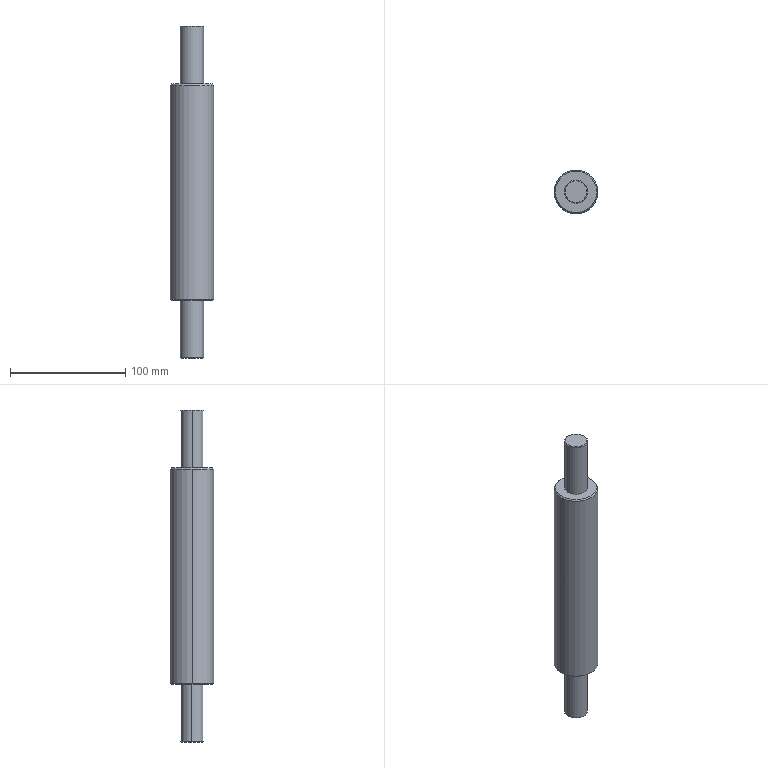Component | SolidWorks | CuttingMotorFixedAxis-1 | 1 solid | 18 faces | box 38 x 38 x 288 mm | volume 244475 mm3 | cone 8 | cylinder 6 | plane 4 | commonest cylinder face diameters 20 x4 38 x2
build123d program:
from build123d import *
from OCP.BRepFilletAPI import BRepFilletAPI_MakeChamfer

# Parameters (mm, degrees)
CHAMFER1_SIZE  = 0.5
CHAMFER2_SIZE  = 1
CHAMFER2_SIZE2 = 1.192


with BuildPart() as part:
    # Sketch1 → Revolve1 (revolve)
    with BuildSketch(Plane.XY, mode=Mode.PRIVATE) as revolve1_sk:
        Polygon((0, 0), (0, 10), (50, 10), (50, 19), (238, 19), (238, 10), (288, 10), (288, 0), align=None)
    revolve(revolve1_sk.sketch.rotate(Axis((-313.729, 0, 0), (1, 0, 0)), 90), axis=Axis((-313.729, 0, 0), (1, 0, 0)))

    # Chamfer1
    chamfer1_edges = [part.edges().sort_by_distance(p)[0] for p in [
        (288, 0, -10),
        (0, 0, -10),
    ]]
    chamfer(chamfer1_edges, length=CHAMFER1_SIZE)

    # Chamfer2: one chamfer whose edges measure the first distance from different faces: ONE call of the kernel's chamfer builder (chamfer() names one face for all edges)
    chamfer2_edges_1 = [part.edges().sort_by_distance(p)[0] for p in [
        (238, 0, -19),
    ]]
    chamfer2_side_1 = [part.faces().sort_by_distance(p)[0] for p in [
        (238, 0, -18.463),
    ]]
    chamfer2_edges_2 = [part.edges().sort_by_distance(p)[0] for p in [
        (50, 0, -19),
    ]]
    chamfer2_side_2 = [part.faces().sort_by_distance(p)[0] for p in [
        (144, 0, -19),
    ]]
    chamfer2 = BRepFilletAPI_MakeChamfer(part.part.solid().wrapped)
    for e in chamfer2_edges_1:
        chamfer2.Add(CHAMFER2_SIZE, CHAMFER2_SIZE2, e.wrapped, chamfer2_side_1[0].wrapped)  # the first distance lies on this face
    for e in chamfer2_edges_2:
        chamfer2.Add(CHAMFER2_SIZE, CHAMFER2_SIZE2, e.wrapped, chamfer2_side_2[0].wrapped)  # the first distance lies on this face
    add(Compound.cast(chamfer2.Shape()), mode=Mode.REPLACE)


solid = part.part

# Placed as in the assembly
solid = solid.moved(Location((-22.772, -46.766, 756), (0, -90, 0)))
STEP:
#1=COLOUR_RGB('',0.7922,0.8196,0.9333);
#2=FILL_AREA_STYLE_COLOUR('',#1);
#3=FILL_AREA_STYLE('',(#2));
#4=SURFACE_STYLE_FILL_AREA(#3);
#5=SURFACE_SIDE_STYLE('',(#4));
#6=SURFACE_STYLE_USAGE(.BOTH.,#5);
#7=PRESENTATION_STYLE_ASSIGNMENT((#6));
#8=CARTESIAN_POINT('',(-1.598,-1.841,31.732));
#9=VERTEX_POINT('',#8);
#10=CARTESIAN_POINT('',(-0.1954,-1.841,31.732));
#11=VERTEX_POINT('',#10);
#12=CARTESIAN_POINT('',(-0.8965,-1.841,31.732));
#13=DIRECTION('',(-0.,0.,-1.));
#14=DIRECTION('',(1.,0.,0.));
#15=AXIS2_PLACEMENT_3D('',#12,#13,#14);
#16=CIRCLE('',#15,0.7011);
#17=EDGE_CURVE('',#9,#11,#16,.T.);
#18=ORIENTED_EDGE('',*,*,#17,.F.);
#19=CARTESIAN_POINT('',(-1.645,-1.841,31.772));
#20=VERTEX_POINT('',#19);
#21=CARTESIAN_POINT('',(-1.598,-1.841,31.732));
#22=DIRECTION('',(-0.766,-0.,0.6428));
#23=VECTOR('',#22,39.37);
#24=LINE('',#21,#23);
#25=EDGE_CURVE('',#9,#20,#24,.T.);
#26=ORIENTED_EDGE('',*,*,#25,.T.);
#27=CARTESIAN_POINT('',(-0.1485,-1.841,31.772));
#28=VERTEX_POINT('',#27);
#29=CARTESIAN_POINT('',(-0.8965,-1.841,31.772));
#30=DIRECTION('',(0.,-0.,1.));
#31=DIRECTION('',(1.,0.,0.));
#32=AXIS2_PLACEMENT_3D('',#29,#30,#31);
#33=CIRCLE('',#32,0.748);
#34=EDGE_CURVE('',#28,#20,#33,.T.);
#35=ORIENTED_EDGE('',*,*,#34,.F.);
#36=CARTESIAN_POINT('',(-0.1954,-1.841,31.732));
#37=DIRECTION('',(0.766,-0.,0.6428));
#38=VECTOR('',#37,39.37);
#39=LINE('',#36,#38);
#40=EDGE_CURVE('',#11,#28,#39,.T.);
#41=ORIENTED_EDGE('',*,*,#40,.F.);
#42=EDGE_LOOP('',(#18,#26,#35,#41));
#43=FACE_OUTER_BOUND('',#42,.T.);
#44=CARTESIAN_POINT('',(-0.8965,-1.841,31.732));
#45=DIRECTION('',(0.,-0.,1.));
#46=DIRECTION('',(1.,0.,0.));
#47=AXIS2_PLACEMENT_3D('',#44,#45,#46);
#48=CONICAL_SURFACE('',#47,0.7011,0.8727);
#49=ADVANCED_FACE('',(#43),#48,.T.);
#50=CARTESIAN_POINT('',(-0.1879,-1.841,39.134));
#51=VERTEX_POINT('',#50);
#52=CARTESIAN_POINT('',(-1.605,-1.841,39.134));
#53=VERTEX_POINT('',#52);
#54=CARTESIAN_POINT('',(-0.8965,-1.841,39.134));
#55=DIRECTION('',(0.,-0.,1.));
#56=DIRECTION('',(-1.,-0.,0.));
#57=AXIS2_PLACEMENT_3D('',#54,#55,#56);
#58=CIRCLE('',#57,0.7087);
#59=EDGE_CURVE('',#51,#53,#58,.T.);
#60=ORIENTED_EDGE('',*,*,#59,.F.);
#61=CARTESIAN_POINT('',(-0.1485,-1.841,39.087));
#62=VERTEX_POINT('',#61);
#63=CARTESIAN_POINT('',(-0.1485,-1.841,39.087));
#64=DIRECTION('',(0.6428,0.,-0.766));
#65=VECTOR('',#64,39.37);
#66=LINE('',#63,#65);
#67=EDGE_CURVE('',#51,#62,#66,.T.);
#68=ORIENTED_EDGE('',*,*,#67,.T.);
#69=CARTESIAN_POINT('',(-1.645,-1.841,39.087));
#70=VERTEX_POINT('',#69);
#71=CARTESIAN_POINT('',(-0.8965,-1.841,39.087));
#72=DIRECTION('',(-0.,0.,-1.));
#73=DIRECTION('',(-1.,-0.,0.));
#74=AXIS2_PLACEMENT_3D('',#71,#72,#73);
#75=CIRCLE('',#74,0.748);
#76=EDGE_CURVE('',#70,#62,#75,.T.);
#77=ORIENTED_EDGE('',*,*,#76,.F.);
#78=CARTESIAN_POINT('',(-1.645,-1.841,39.087));
#79=DIRECTION('',(-0.6428,0.,-0.766));
#80=VECTOR('',#79,39.37);
#81=LINE('',#78,#80);
#82=EDGE_CURVE('',#53,#70,#81,.T.);
#83=ORIENTED_EDGE('',*,*,#82,.F.);
#84=EDGE_LOOP('',(#60,#68,#77,#83));
#85=FACE_OUTER_BOUND('',#84,.T.);
#86=CARTESIAN_POINT('',(-0.8965,-1.841,39.087));
#87=DIRECTION('',(-0.,0.,-1.));
#88=DIRECTION('',(-1.,-0.,0.));
#89=AXIS2_PLACEMENT_3D('',#86,#87,#88);
#90=CONICAL_SURFACE('',#89,0.748,0.6981);
#91=ADVANCED_FACE('',(#85),#90,.T.);
#92=CARTESIAN_POINT('',(-1.271,-1.841,29.764));
#93=VERTEX_POINT('',#92);
#94=CARTESIAN_POINT('',(-0.5225,-1.841,29.764));
#95=VERTEX_POINT('',#94);
#96=CARTESIAN_POINT('',(-0.8965,-1.841,29.764));
#97=DIRECTION('',(-0.,0.,-1.));
#98=DIRECTION('',(1.,0.,0.));
#99=AXIS2_PLACEMENT_3D('',#96,#97,#98);
#100=CIRCLE('',#99,0.374);
#101=EDGE_CURVE('',#93,#95,#100,.T.);
#102=ORIENTED_EDGE('',*,*,#101,.F.);
#103=CARTESIAN_POINT('',(-1.29,-1.841,29.783));
#104=VERTEX_POINT('',#103);
#105=CARTESIAN_POINT('',(-1.271,-1.841,29.764));
#106=DIRECTION('',(-0.7071,-0.,0.7071));
#107=VECTOR('',#106,39.37);
#108=LINE('',#105,#107);
#109=EDGE_CURVE('',#93,#104,#108,.T.);
#110=ORIENTED_EDGE('',*,*,#109,.T.);
#111=CARTESIAN_POINT('',(-0.5028,-1.841,29.783));
#112=VERTEX_POINT('',#111);
#113=CARTESIAN_POINT('',(-0.8965,-1.841,29.783));
#114=DIRECTION('',(0.,-0.,1.));
#115=DIRECTION('',(1.,0.,0.));
#116=AXIS2_PLACEMENT_3D('',#113,#114,#115);
#117=CIRCLE('',#116,0.3937);
#118=EDGE_CURVE('',#112,#104,#117,.T.);
#119=ORIENTED_EDGE('',*,*,#118,.F.);
#120=CARTESIAN_POINT('',(-0.5225,-1.841,29.764));
#121=DIRECTION('',(0.7071,-0.,0.7071));
#122=VECTOR('',#121,39.37);
#123=LINE('',#120,#122);
#124=EDGE_CURVE('',#95,#112,#123,.T.);
#125=ORIENTED_EDGE('',*,*,#124,.F.);
#126=EDGE_LOOP('',(#102,#110,#119,#125));
#127=FACE_OUTER_BOUND('',#126,.T.);
#128=CARTESIAN_POINT('',(-0.8965,-1.841,29.764));
#129=DIRECTION('',(0.,-0.,1.));
#130=DIRECTION('',(1.,0.,0.));
#131=AXIS2_PLACEMENT_3D('',#128,#129,#130);
#132=CONICAL_SURFACE('',#131,0.374,0.7854);
#133=ADVANCED_FACE('',(#127),#132,.T.);
#134=CARTESIAN_POINT('',(-0.5225,-1.841,41.102));
#135=VERTEX_POINT('',#134);
#136=CARTESIAN_POINT('',(-1.271,-1.841,41.102));
#137=VERTEX_POINT('',#136);
#138=CARTESIAN_POINT('',(-0.8965,-1.841,41.102));
#139=DIRECTION('',(0.,-0.,1.));
#140=DIRECTION('',(-1.,0.,0.));
#141=AXIS2_PLACEMENT_3D('',#138,#139,#140);
#142=CIRCLE('',#141,0.374);
#143=EDGE_CURVE('',#135,#137,#142,.T.);
#144=ORIENTED_EDGE('',*,*,#143,.F.);
#145=CARTESIAN_POINT('',(-0.5028,-1.841,41.083));
#146=VERTEX_POINT('',#145);
#147=CARTESIAN_POINT('',(-0.5028,-1.841,41.083));
#148=DIRECTION('',(0.7071,0.,-0.7071));
#149=VECTOR('',#148,39.37);
#150=LINE('',#147,#149);
#151=EDGE_CURVE('',#135,#146,#150,.T.);
#152=ORIENTED_EDGE('',*,*,#151,.T.);
#153=CARTESIAN_POINT('',(-1.29,-1.841,41.083));
#154=VERTEX_POINT('',#153);
#155=CARTESIAN_POINT('',(-0.8965,-1.841,41.083));
#156=DIRECTION('',(-0.,0.,-1.));
#157=DIRECTION('',(-1.,0.,0.));
#158=AXIS2_PLACEMENT_3D('',#155,#156,#157);
#159=CIRCLE('',#158,0.3937);
#160=EDGE_CURVE('',#154,#146,#159,.T.);
#161=ORIENTED_EDGE('',*,*,#160,.F.);
#162=CARTESIAN_POINT('',(-1.29,-1.841,41.083));
#163=DIRECTION('',(-0.7071,0.,-0.7071));
#164=VECTOR('',#163,39.37);
#165=LINE('',#162,#164);
#166=EDGE_CURVE('',#137,#154,#165,.T.);
#167=ORIENTED_EDGE('',*,*,#166,.F.);
#168=EDGE_LOOP('',(#144,#152,#161,#167));
#169=FACE_OUTER_BOUND('',#168,.T.);
#170=CARTESIAN_POINT('',(-0.8965,-1.841,41.083));
#171=DIRECTION('',(-0.,0.,-1.));
#172=DIRECTION('',(-1.,0.,0.));
#173=AXIS2_PLACEMENT_3D('',#170,#171,#172);
#174=CONICAL_SURFACE('',#173,0.3937,0.7854);
#175=ADVANCED_FACE('',(#169),#174,.T.);
#176=ORIENTED_EDGE('',*,*,#160,.T.);
#177=CARTESIAN_POINT('',(-0.5028,-1.841,39.134));
#178=VERTEX_POINT('',#177);
#179=CARTESIAN_POINT('',(-0.5028,-1.841,17.412));
#180=DIRECTION('',(-0.,0.,-1.));
#181=VECTOR('',#180,39.37);
#182=LINE('',#179,#181);
#183=EDGE_CURVE('',#146,#178,#182,.T.);
#184=ORIENTED_EDGE('',*,*,#183,.T.);
#185=CARTESIAN_POINT('',(-1.29,-1.841,39.134));
#186=VERTEX_POINT('',#185);
#187=CARTESIAN_POINT('',(-0.8965,-1.841,39.134));
#188=DIRECTION('',(-0.,0.,-1.));
#189=DIRECTION('',(-1.,0.,0.));
#190=AXIS2_PLACEMENT_3D('',#187,#188,#189);
#191=CIRCLE('',#190,0.3937);
#192=EDGE_CURVE('',#186,#178,#191,.T.);
#193=ORIENTED_EDGE('',*,*,#192,.F.);
#194=CARTESIAN_POINT('',(-1.29,-1.841,17.412));
#195=DIRECTION('',(-0.,0.,-1.));
#196=VECTOR('',#195,39.37);
#197=LINE('',#194,#196);
#198=EDGE_CURVE('',#154,#186,#197,.T.);
#199=ORIENTED_EDGE('',*,*,#198,.F.);
#200=EDGE_LOOP('',(#176,#184,#193,#199));
#201=FACE_OUTER_BOUND('',#200,.T.);
#202=CARTESIAN_POINT('',(-0.8965,-1.841,17.412));
#203=DIRECTION('',(-0.,0.,-1.));
#204=DIRECTION('',(-1.,0.,0.));
#205=AXIS2_PLACEMENT_3D('',#202,#203,#204);
#206=CYLINDRICAL_SURFACE('',#205,0.3937);
#207=ADVANCED_FACE('',(#201),#206,.T.);
#208=ORIENTED_EDGE('',*,*,#76,.T.);
#209=CARTESIAN_POINT('',(-0.1485,-1.841,17.412));
#210=DIRECTION('',(-0.,0.,-1.));
#211=VECTOR('',#210,39.37);
#212=LINE('',#209,#211);
#213=EDGE_CURVE('',#62,#28,#212,.T.);
#214=ORIENTED_EDGE('',*,*,#213,.T.);
#215=ORIENTED_EDGE('',*,*,#34,.T.);
#216=CARTESIAN_POINT('',(-1.645,-1.841,17.412));
#217=DIRECTION('',(-0.,0.,-1.));
#218=VECTOR('',#217,39.37);
#219=LINE('',#216,#218);
#220=EDGE_CURVE('',#70,#20,#219,.T.);
#221=ORIENTED_EDGE('',*,*,#220,.F.);
#222=EDGE_LOOP('',(#208,#214,#215,#221));
#223=FACE_OUTER_BOUND('',#222,.T.);
#224=CARTESIAN_POINT('',(-0.8965,-1.841,17.412));
#225=DIRECTION('',(-0.,0.,-1.));
#226=DIRECTION('',(-1.,-0.,0.));
#227=AXIS2_PLACEMENT_3D('',#224,#225,#226);
#228=CYLINDRICAL_SURFACE('',#227,0.748);
#229=ADVANCED_FACE('',(#223),#228,.T.);
#230=CARTESIAN_POINT('',(-1.29,-1.841,31.732));
#231=VERTEX_POINT('',#230);
#232=CARTESIAN_POINT('',(-0.5028,-1.841,31.732));
#233=VERTEX_POINT('',#232);
#234=CARTESIAN_POINT('',(-0.8965,-1.841,31.732));
#235=DIRECTION('',(-0.,0.,-1.));
#236=DIRECTION('',(-1.,0.,0.));
#237=AXIS2_PLACEMENT_3D('',#234,#235,#236);
#238=CIRCLE('',#237,0.3937);
#239=EDGE_CURVE('',#231,#233,#238,.T.);
#240=ORIENTED_EDGE('',*,*,#239,.T.);
#241=CARTESIAN_POINT('',(-0.5028,-1.841,17.412));
#242=DIRECTION('',(-0.,0.,-1.));
#243=VECTOR('',#242,39.37);
#244=LINE('',#241,#243);
#245=EDGE_CURVE('',#233,#112,#244,.T.);
#246=ORIENTED_EDGE('',*,*,#245,.T.);
#247=ORIENTED_EDGE('',*,*,#118,.T.);
#248=CARTESIAN_POINT('',(-1.29,-1.841,17.412));
#249=DIRECTION('',(-0.,0.,-1.));
#250=VECTOR('',#249,39.37);
#251=LINE('',#248,#250);
#252=EDGE_CURVE('',#231,#104,#251,.T.);
#253=ORIENTED_EDGE('',*,*,#252,.F.);
#254=EDGE_LOOP('',(#240,#246,#247,#253));
#255=FACE_OUTER_BOUND('',#254,.T.);
#256=CARTESIAN_POINT('',(-0.8965,-1.841,17.412));
#257=DIRECTION('',(-0.,0.,-1.));
#258=DIRECTION('',(-1.,0.,0.));
#259=AXIS2_PLACEMENT_3D('',#256,#257,#258);
#260=CYLINDRICAL_SURFACE('',#259,0.3937);
#261=ADVANCED_FACE('',(#255),#260,.T.);
#262=CARTESIAN_POINT('',(-0.8965,-1.841,29.764));
#263=DIRECTION('',(-0.,0.,-1.));
#264=DIRECTION('',(1.,0.,0.));
#265=AXIS2_PLACEMENT_3D('',#262,#263,#264);
#266=CIRCLE('',#265,0.374);
#267=EDGE_CURVE('',#95,#93,#266,.T.);
#268=ORIENTED_EDGE('',*,*,#267,.T.);
#269=ORIENTED_EDGE('',*,*,#101,.T.);
#270=EDGE_LOOP('',(#268,#269));
#271=FACE_OUTER_BOUND('',#270,.T.);
#272=CARTESIAN_POINT('',(-0.8965,-1.841,29.764));
#273=DIRECTION('',(0.,-0.,1.));
#274=DIRECTION('',(1.,0.,-0.));
#275=AXIS2_PLACEMENT_3D('',#272,#273,#274);
#276=PLANE('',#275);
#277=ADVANCED_FACE('',(#271),#276,.F.);
#278=ORIENTED_EDGE('',*,*,#245,.F.);
#279=CARTESIAN_POINT('',(-0.8965,-1.841,31.732));
#280=DIRECTION('',(-0.,0.,-1.));
#281=DIRECTION('',(-1.,0.,0.));
#282=AXIS2_PLACEMENT_3D('',#279,#280,#281);
#283=CIRCLE('',#282,0.3937);
#284=EDGE_CURVE('',#233,#231,#283,.T.);
#285=ORIENTED_EDGE('',*,*,#284,.T.);
#286=ORIENTED_EDGE('',*,*,#252,.T.);
#287=CARTESIAN_POINT('',(-0.8965,-1.841,29.783));
#288=DIRECTION('',(0.,-0.,1.));
#289=DIRECTION('',(1.,0.,0.));
#290=AXIS2_PLACEMENT_3D('',#287,#288,#289);
#291=CIRCLE('',#290,0.3937);
#292=EDGE_CURVE('',#104,#112,#291,.T.);
#293=ORIENTED_EDGE('',*,*,#292,.T.);
#294=EDGE_LOOP('',(#278,#285,#286,#293));
#295=FACE_OUTER_BOUND('',#294,.T.);
#296=CARTESIAN_POINT('',(-0.8965,-1.841,17.412));
#297=DIRECTION('',(-0.,0.,-1.));
#298=DIRECTION('',(-1.,0.,0.));
#299=AXIS2_PLACEMENT_3D('',#296,#297,#298);
#300=CYLINDRICAL_SURFACE('',#299,0.3937);
#301=ADVANCED_FACE('',(#295),#300,.T.);
#302=CARTESIAN_POINT('',(-0.8965,-1.841,31.732));
#303=DIRECTION('',(-0.,0.,-1.));
#304=DIRECTION('',(1.,0.,0.));
#305=AXIS2_PLACEMENT_3D('',#302,#303,#304);
#306=CIRCLE('',#305,0.7011);
#307=EDGE_CURVE('',#11,#9,#306,.T.);
#308=ORIENTED_EDGE('',*,*,#307,.T.);
#309=ORIENTED_EDGE('',*,*,#17,.T.);
#310=EDGE_LOOP('',(#308,#309));
#311=FACE_OUTER_BOUND('',#310,.T.);
#312=ORIENTED_EDGE('',*,*,#239,.F.);
#313=ORIENTED_EDGE('',*,*,#284,.F.);
#314=EDGE_LOOP('',(#312,#313));
#315=FACE_BOUND('',#314,.T.);
#316=CARTESIAN_POINT('',(-0.8965,-1.447,31.732));
#317=DIRECTION('',(0.,-0.,1.));
#318=DIRECTION('',(1.,0.,-0.));
#319=AXIS2_PLACEMENT_3D('',#316,#317,#318);
#320=PLANE('',#319);
#321=ADVANCED_FACE('',(#311,#315),#320,.F.);
#322=ORIENTED_EDGE('',*,*,#213,.F.);
#323=CARTESIAN_POINT('',(-0.8965,-1.841,39.087));
#324=DIRECTION('',(-0.,0.,-1.));
#325=DIRECTION('',(-1.,-0.,0.));
#326=AXIS2_PLACEMENT_3D('',#323,#324,#325);
#327=CIRCLE('',#326,0.748);
#328=EDGE_CURVE('',#62,#70,#327,.T.);
#329=ORIENTED_EDGE('',*,*,#328,.T.);
#330=ORIENTED_EDGE('',*,*,#220,.T.);
#331=CARTESIAN_POINT('',(-0.8965,-1.841,31.772));
#332=DIRECTION('',(0.,-0.,1.));
#333=DIRECTION('',(1.,0.,0.));
#334=AXIS2_PLACEMENT_3D('',#331,#332,#333);
#335=CIRCLE('',#334,0.748);
#336=EDGE_CURVE('',#20,#28,#335,.T.);
#337=ORIENTED_EDGE('',*,*,#336,.T.);
#338=EDGE_LOOP('',(#322,#329,#330,#337));
#339=FACE_OUTER_BOUND('',#338,.T.);
#340=CARTESIAN_POINT('',(-0.8965,-1.841,17.412));
#341=DIRECTION('',(-0.,0.,-1.));
#342=DIRECTION('',(-1.,-0.,0.));
#343=AXIS2_PLACEMENT_3D('',#340,#341,#342);
#344=CYLINDRICAL_SURFACE('',#343,0.748);
#345=ADVANCED_FACE('',(#339),#344,.T.);
#346=CARTESIAN_POINT('',(-0.8965,-1.841,39.134));
#347=DIRECTION('',(0.,-0.,1.));
#348=DIRECTION('',(-1.,-0.,0.));
#349=AXIS2_PLACEMENT_3D('',#346,#347,#348);
#350=CIRCLE('',#349,0.7087);
#351=EDGE_CURVE('',#53,#51,#350,.T.);
#352=ORIENTED_EDGE('',*,*,#351,.T.);
#353=ORIENTED_EDGE('',*,*,#59,.T.);
#354=EDGE_LOOP('',(#352,#353));
#355=FACE_OUTER_BOUND('',#354,.T.);
#356=ORIENTED_EDGE('',*,*,#192,.T.);
#357=CARTESIAN_POINT('',(-0.8965,-1.841,39.134));
#358=DIRECTION('',(-0.,0.,-1.));
#359=DIRECTION('',(-1.,0.,0.));
#360=AXIS2_PLACEMENT_3D('',#357,#358,#359);
#361=CIRCLE('',#360,0.3937);
#362=EDGE_CURVE('',#178,#186,#361,.T.);
#363=ORIENTED_EDGE('',*,*,#362,.T.);
#364=EDGE_LOOP('',(#356,#363));
#365=FACE_BOUND('',#364,.T.);
#366=CARTESIAN_POINT('',(-0.8965,-1.093,39.134));
#367=DIRECTION('',(-0.,0.,-1.));
#368=DIRECTION('',(-1.,-0.,0.));
#369=AXIS2_PLACEMENT_3D('',#366,#367,#368);
#370=PLANE('',#369);
#371=ADVANCED_FACE('',(#355,#365),#370,.F.);
#372=ORIENTED_EDGE('',*,*,#183,.F.);
#373=CARTESIAN_POINT('',(-0.8965,-1.841,41.083));
#374=DIRECTION('',(-0.,0.,-1.));
#375=DIRECTION('',(-1.,0.,0.));
#376=AXIS2_PLACEMENT_3D('',#373,#374,#375);
#377=CIRCLE('',#376,0.3937);
#378=EDGE_CURVE('',#146,#154,#377,.T.);
#379=ORIENTED_EDGE('',*,*,#378,.T.);
#380=ORIENTED_EDGE('',*,*,#198,.T.);
#381=ORIENTED_EDGE('',*,*,#362,.F.);
#382=EDGE_LOOP('',(#372,#379,#380,#381));
#383=FACE_OUTER_BOUND('',#382,.T.);
#384=CARTESIAN_POINT('',(-0.8965,-1.841,17.412));
#385=DIRECTION('',(-0.,0.,-1.));
#386=DIRECTION('',(-1.,0.,0.));
#387=AXIS2_PLACEMENT_3D('',#384,#385,#386);
#388=CYLINDRICAL_SURFACE('',#387,0.3937);
#389=ADVANCED_FACE('',(#383),#388,.T.);
#390=CARTESIAN_POINT('',(-0.8965,-1.841,41.102));
#391=DIRECTION('',(0.,-0.,1.));
#392=DIRECTION('',(-1.,0.,0.));
#393=AXIS2_PLACEMENT_3D('',#390,#391,#392);
#394=CIRCLE('',#393,0.374);
#395=EDGE_CURVE('',#137,#135,#394,.T.);
#396=ORIENTED_EDGE('',*,*,#395,.T.);
#397=ORIENTED_EDGE('',*,*,#143,.T.);
#398=EDGE_LOOP('',(#396,#397));
#399=FACE_OUTER_BOUND('',#398,.T.);
#400=CARTESIAN_POINT('',(-0.8965,-1.447,41.102));
#401=DIRECTION('',(-0.,0.,-1.));
#402=DIRECTION('',(-1.,-0.,0.));
#403=AXIS2_PLACEMENT_3D('',#400,#401,#402);
#404=PLANE('',#403);
#405=ADVANCED_FACE('',(#399),#404,.F.);
#406=ORIENTED_EDGE('',*,*,#151,.F.);
#407=ORIENTED_EDGE('',*,*,#395,.F.);
#408=ORIENTED_EDGE('',*,*,#166,.T.);
#409=ORIENTED_EDGE('',*,*,#378,.F.);
#410=EDGE_LOOP('',(#406,#407,#408,#409));
#411=FACE_OUTER_BOUND('',#410,.T.);
#412=CARTESIAN_POINT('',(-0.8965,-1.841,41.083));
#413=DIRECTION('',(-0.,0.,-1.));
#414=DIRECTION('',(-1.,0.,0.));
#415=AXIS2_PLACEMENT_3D('',#412,#413,#414);
#416=CONICAL_SURFACE('',#415,0.3937,0.7854);
#417=ADVANCED_FACE('',(#411),#416,.T.);
#418=ORIENTED_EDGE('',*,*,#109,.F.);
#419=ORIENTED_EDGE('',*,*,#267,.F.);
#420=ORIENTED_EDGE('',*,*,#124,.T.);
#421=ORIENTED_EDGE('',*,*,#292,.F.);
#422=EDGE_LOOP('',(#418,#419,#420,#421));
#423=FACE_OUTER_BOUND('',#422,.T.);
#424=CARTESIAN_POINT('',(-0.8965,-1.841,29.764));
#425=DIRECTION('',(0.,-0.,1.));
#426=DIRECTION('',(1.,0.,0.));
#427=AXIS2_PLACEMENT_3D('',#424,#425,#426);
#428=CONICAL_SURFACE('',#427,0.374,0.7854);
#429=ADVANCED_FACE('',(#423),#428,.T.);
#430=ORIENTED_EDGE('',*,*,#67,.F.);
#431=ORIENTED_EDGE('',*,*,#351,.F.);
#432=ORIENTED_EDGE('',*,*,#82,.T.);
#433=ORIENTED_EDGE('',*,*,#328,.F.);
#434=EDGE_LOOP('',(#430,#431,#432,#433));
#435=FACE_OUTER_BOUND('',#434,.T.);
#436=CARTESIAN_POINT('',(-0.8965,-1.841,39.087));
#437=DIRECTION('',(-0.,0.,-1.));
#438=DIRECTION('',(-1.,-0.,0.));
#439=AXIS2_PLACEMENT_3D('',#436,#437,#438);
#440=CONICAL_SURFACE('',#439,0.748,0.6981);
#441=ADVANCED_FACE('',(#435),#440,.T.);
#442=ORIENTED_EDGE('',*,*,#25,.F.);
#443=ORIENTED_EDGE('',*,*,#307,.F.);
#444=ORIENTED_EDGE('',*,*,#40,.T.);
#445=ORIENTED_EDGE('',*,*,#336,.F.);
#446=EDGE_LOOP('',(#442,#443,#444,#445));
#447=FACE_OUTER_BOUND('',#446,.T.);
#448=CARTESIAN_POINT('',(-0.8965,-1.841,31.732));
#449=DIRECTION('',(0.,-0.,1.));
#450=DIRECTION('',(1.,0.,0.));
#451=AXIS2_PLACEMENT_3D('',#448,#449,#450);
#452=CONICAL_SURFACE('',#451,0.7011,0.8727);
#453=ADVANCED_FACE('',(#447),#452,.T.);
#454=CLOSED_SHELL('',(#49,#91,#133,#175,#207,#229,#261,#277,#301,#321,#345,#371,#389,#405,#417,#429,#441,#453));
#455=MANIFOLD_SOLID_BREP('',#454);
#456=STYLED_ITEM('',(#7),#455);
#457=(LENGTH_UNIT()NAMED_UNIT(*)SI_UNIT($,.METRE.));
#458=LENGTH_MEASURE_WITH_UNIT(LENGTH_MEASURE(0.0254),#457);
#459=DIMENSIONAL_EXPONENTS(1.,0.,0.,0.,0.,0.,0.);
#460=(CONVERSION_BASED_UNIT('',#458)LENGTH_UNIT()NAMED_UNIT(#459));
#461=UNCERTAINTY_MEASURE_WITH_UNIT(LENGTH_MEASURE(0.00001),#460,'','');
#462=(NAMED_UNIT(*)PLANE_ANGLE_UNIT()SI_UNIT($,.RADIAN.));
#463=(NAMED_UNIT(*)SI_UNIT($,.STERADIAN.)SOLID_ANGLE_UNIT());
#464=(GEOMETRIC_REPRESENTATION_CONTEXT(3)GLOBAL_UNCERTAINTY_ASSIGNED_CONTEXT((#461))GLOBAL_UNIT_ASSIGNED_CONTEXT((#460,#462,#463))REPRESENTATION_CONTEXT('',''));
#465=MECHANICAL_DESIGN_GEOMETRIC_PRESENTATION_REPRESENTATION('',(#456),#464);
#466=CARTESIAN_POINT('',(0.,0.,0.));
#467=DIRECTION('',(0.,0.,1.));
#468=DIRECTION('',(1.,0.,0.));
#469=AXIS2_PLACEMENT_3D('',#466,#467,#468);
#470=(LENGTH_UNIT()NAMED_UNIT(*)SI_UNIT($,.METRE.));
#471=LENGTH_MEASURE_WITH_UNIT(LENGTH_MEASURE(0.0254),#470);
#472=DIMENSIONAL_EXPONENTS(1.,0.,0.,0.,0.,0.,0.);
#473=(CONVERSION_BASED_UNIT('',#471)LENGTH_UNIT()NAMED_UNIT(#472));
#474=UNCERTAINTY_MEASURE_WITH_UNIT(LENGTH_MEASURE(0.00001),#473,'','');
#475=(NAMED_UNIT(*)PLANE_ANGLE_UNIT()SI_UNIT($,.RADIAN.));
#476=(NAMED_UNIT(*)SI_UNIT($,.STERADIAN.)SOLID_ANGLE_UNIT());
#477=(GEOMETRIC_REPRESENTATION_CONTEXT(3)GLOBAL_UNCERTAINTY_ASSIGNED_CONTEXT((#474))GLOBAL_UNIT_ASSIGNED_CONTEXT((#473,#475,#476))REPRESENTATION_CONTEXT('',''));
#478=ADVANCED_BREP_SHAPE_REPRESENTATION('',(#455,#469),#477);
#479=PRESENTATION_LAYER_ASSIGNMENT('','',(#456));